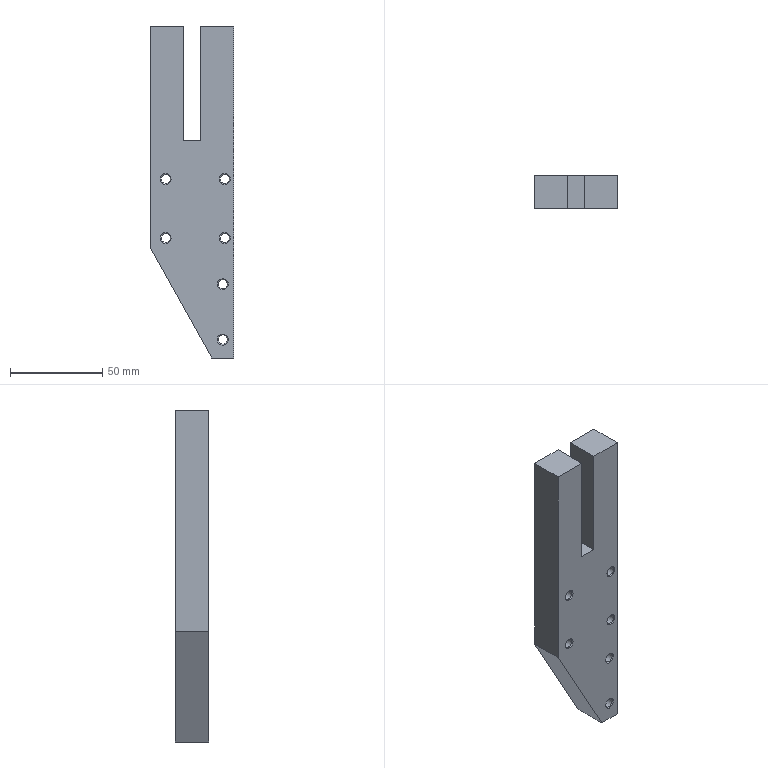Component | NX | AUX_GRIPPER_JAW_VERT_PLATE | 1 solid | 29 faces | volume 116424 mm3 | cone 12 | plane 11 | cylinder 6 | commonest cylinder face diameters 5 x6